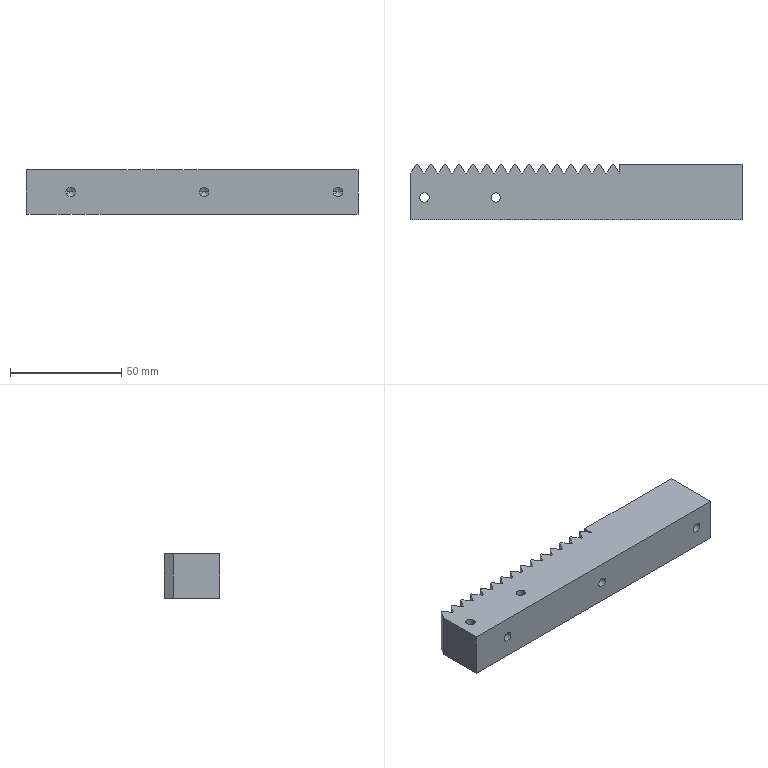Component | SolidWorks | RackAModule2.0-1 | 1 solid | 84 faces | volume 69594 mm3 | plane 68 | cylinder 10 | cone 6 | commonest cylinder face diameters 4.2 x10